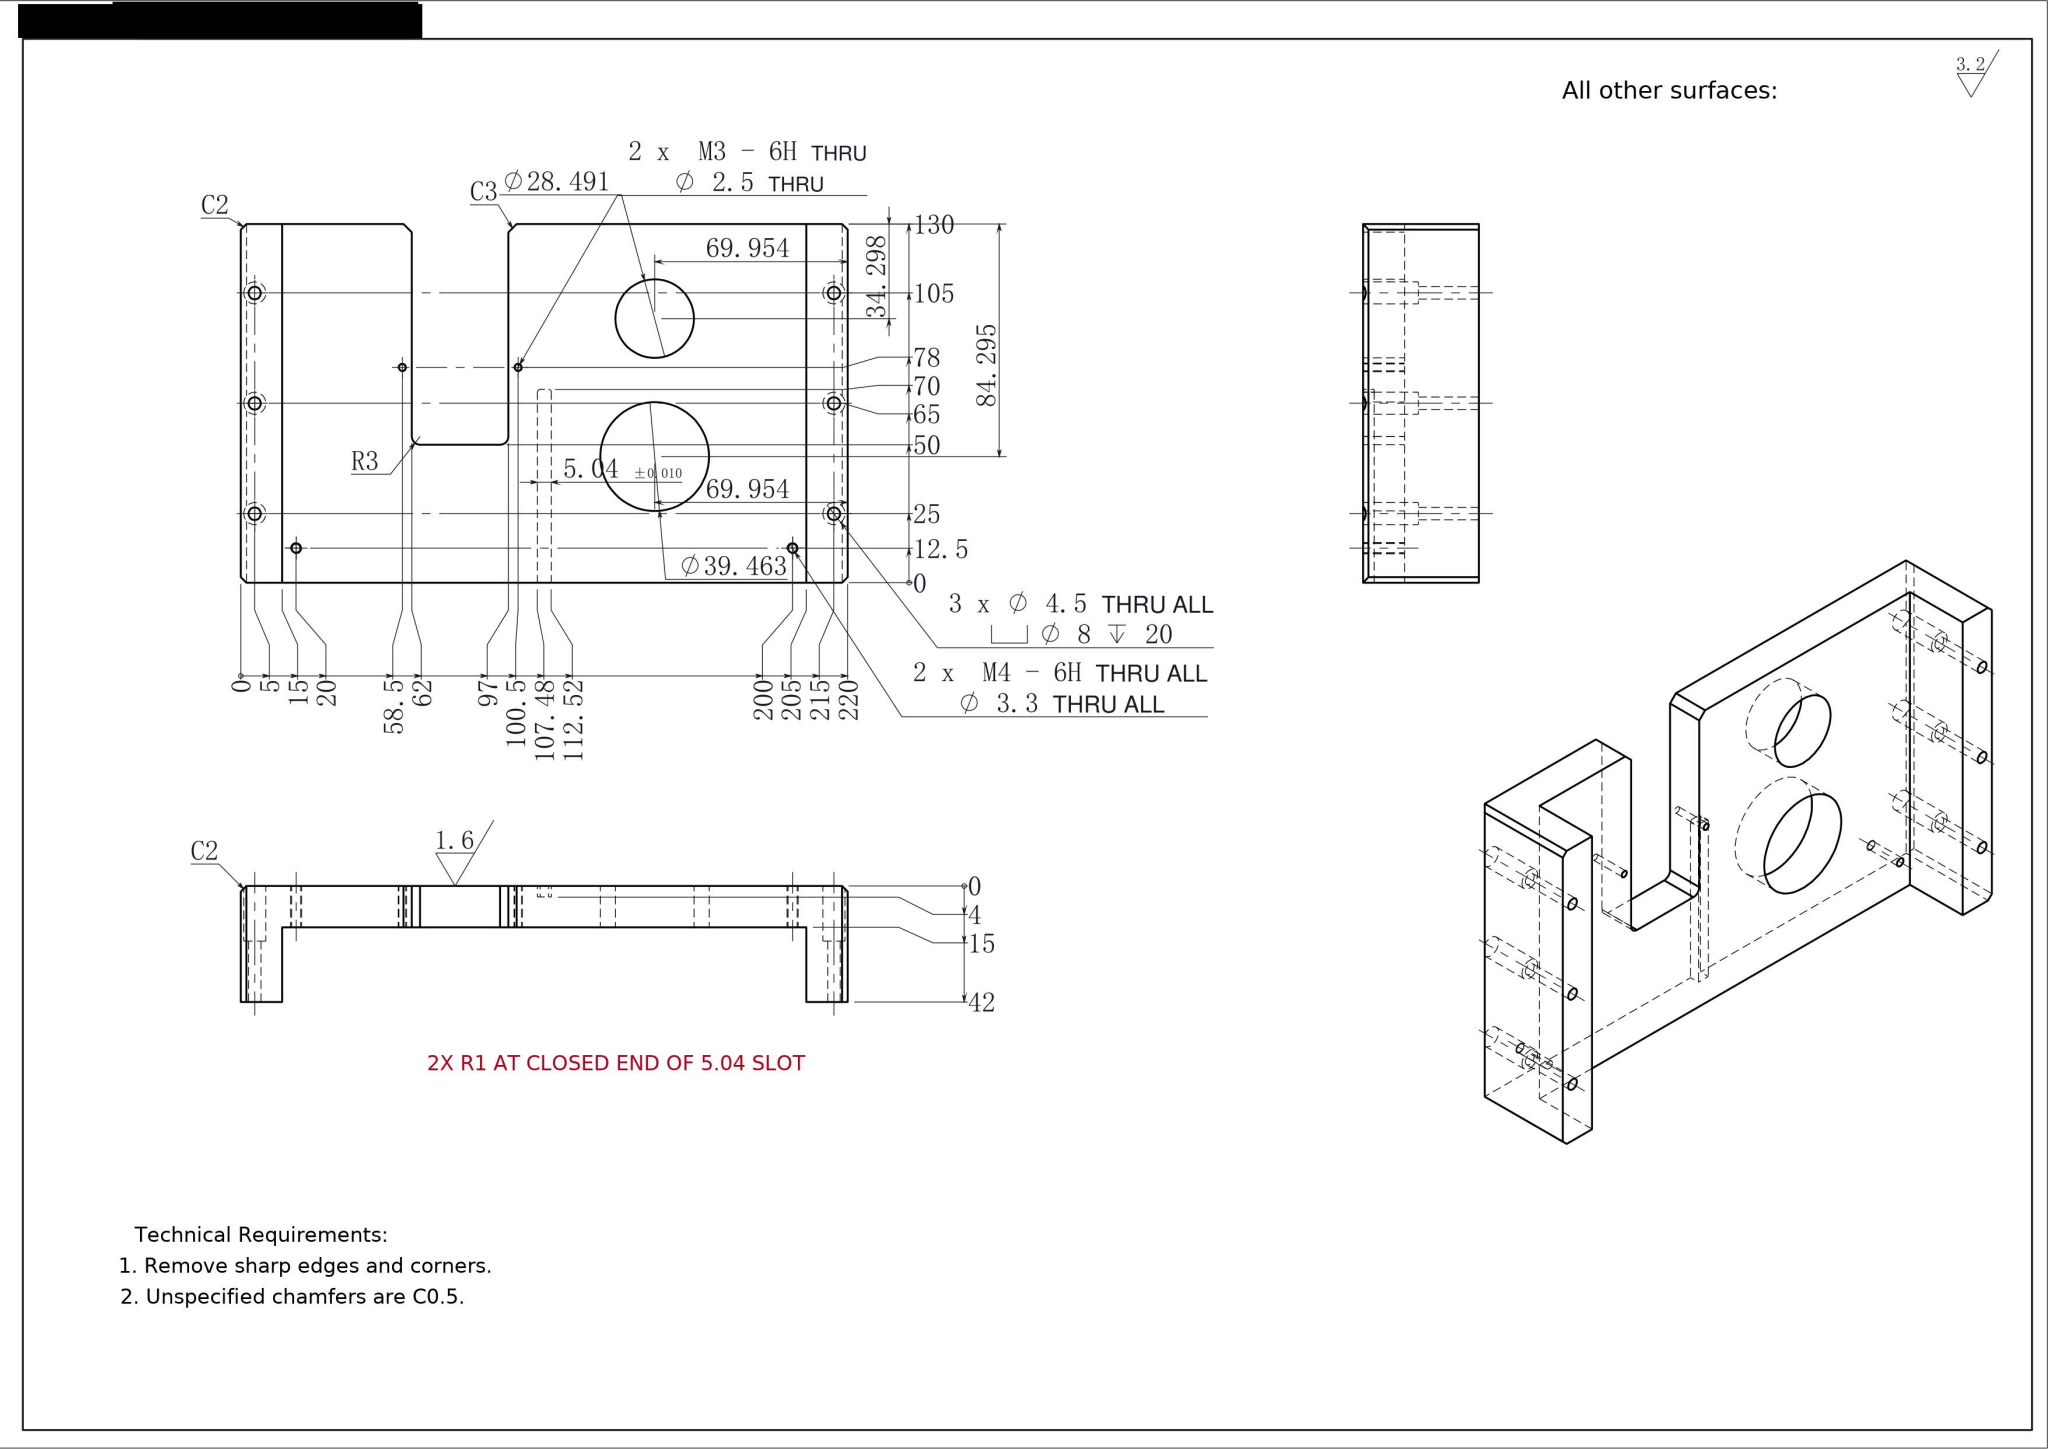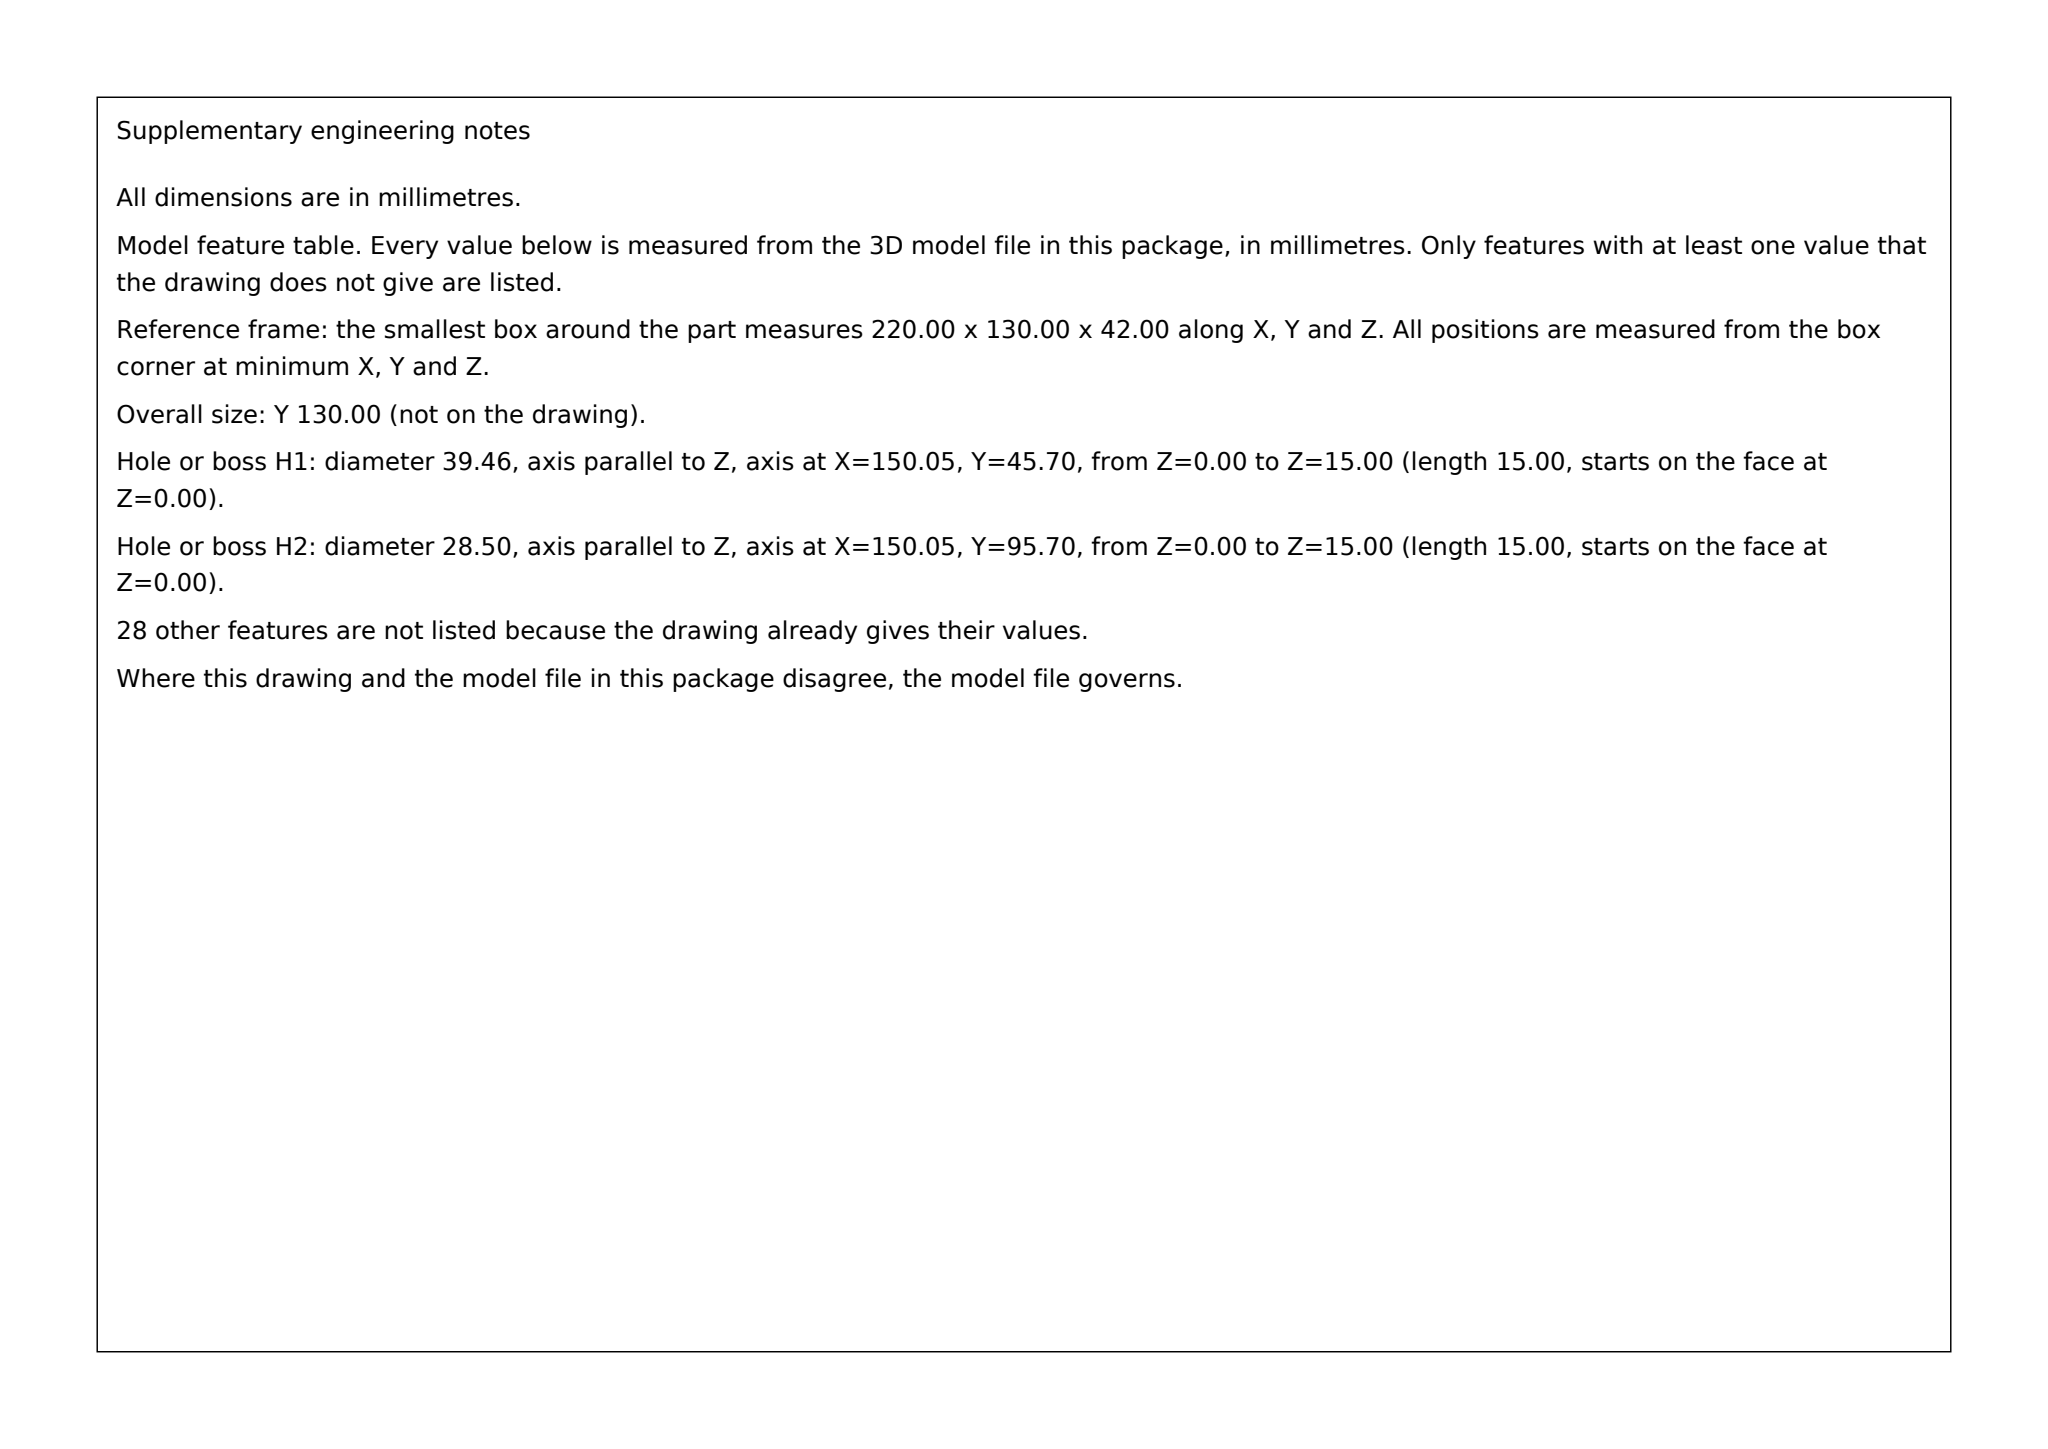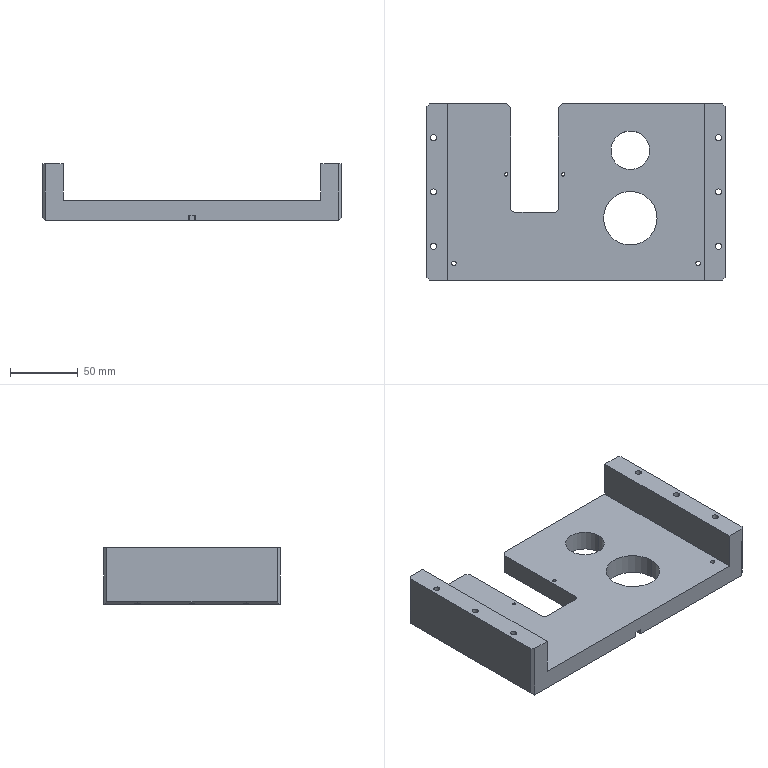Part | SolidWorks | mm | 1 solid | 72 faces | box 220 x 130 x 42 mm | volume 453532 mm3 | cylinder 40 | plane 32 | commonest cylinder face diameters 8 x12 4.5 x12 2.5 x4 3.3 x4 39.463 x2 28.491 x2 6 x2 2 x2